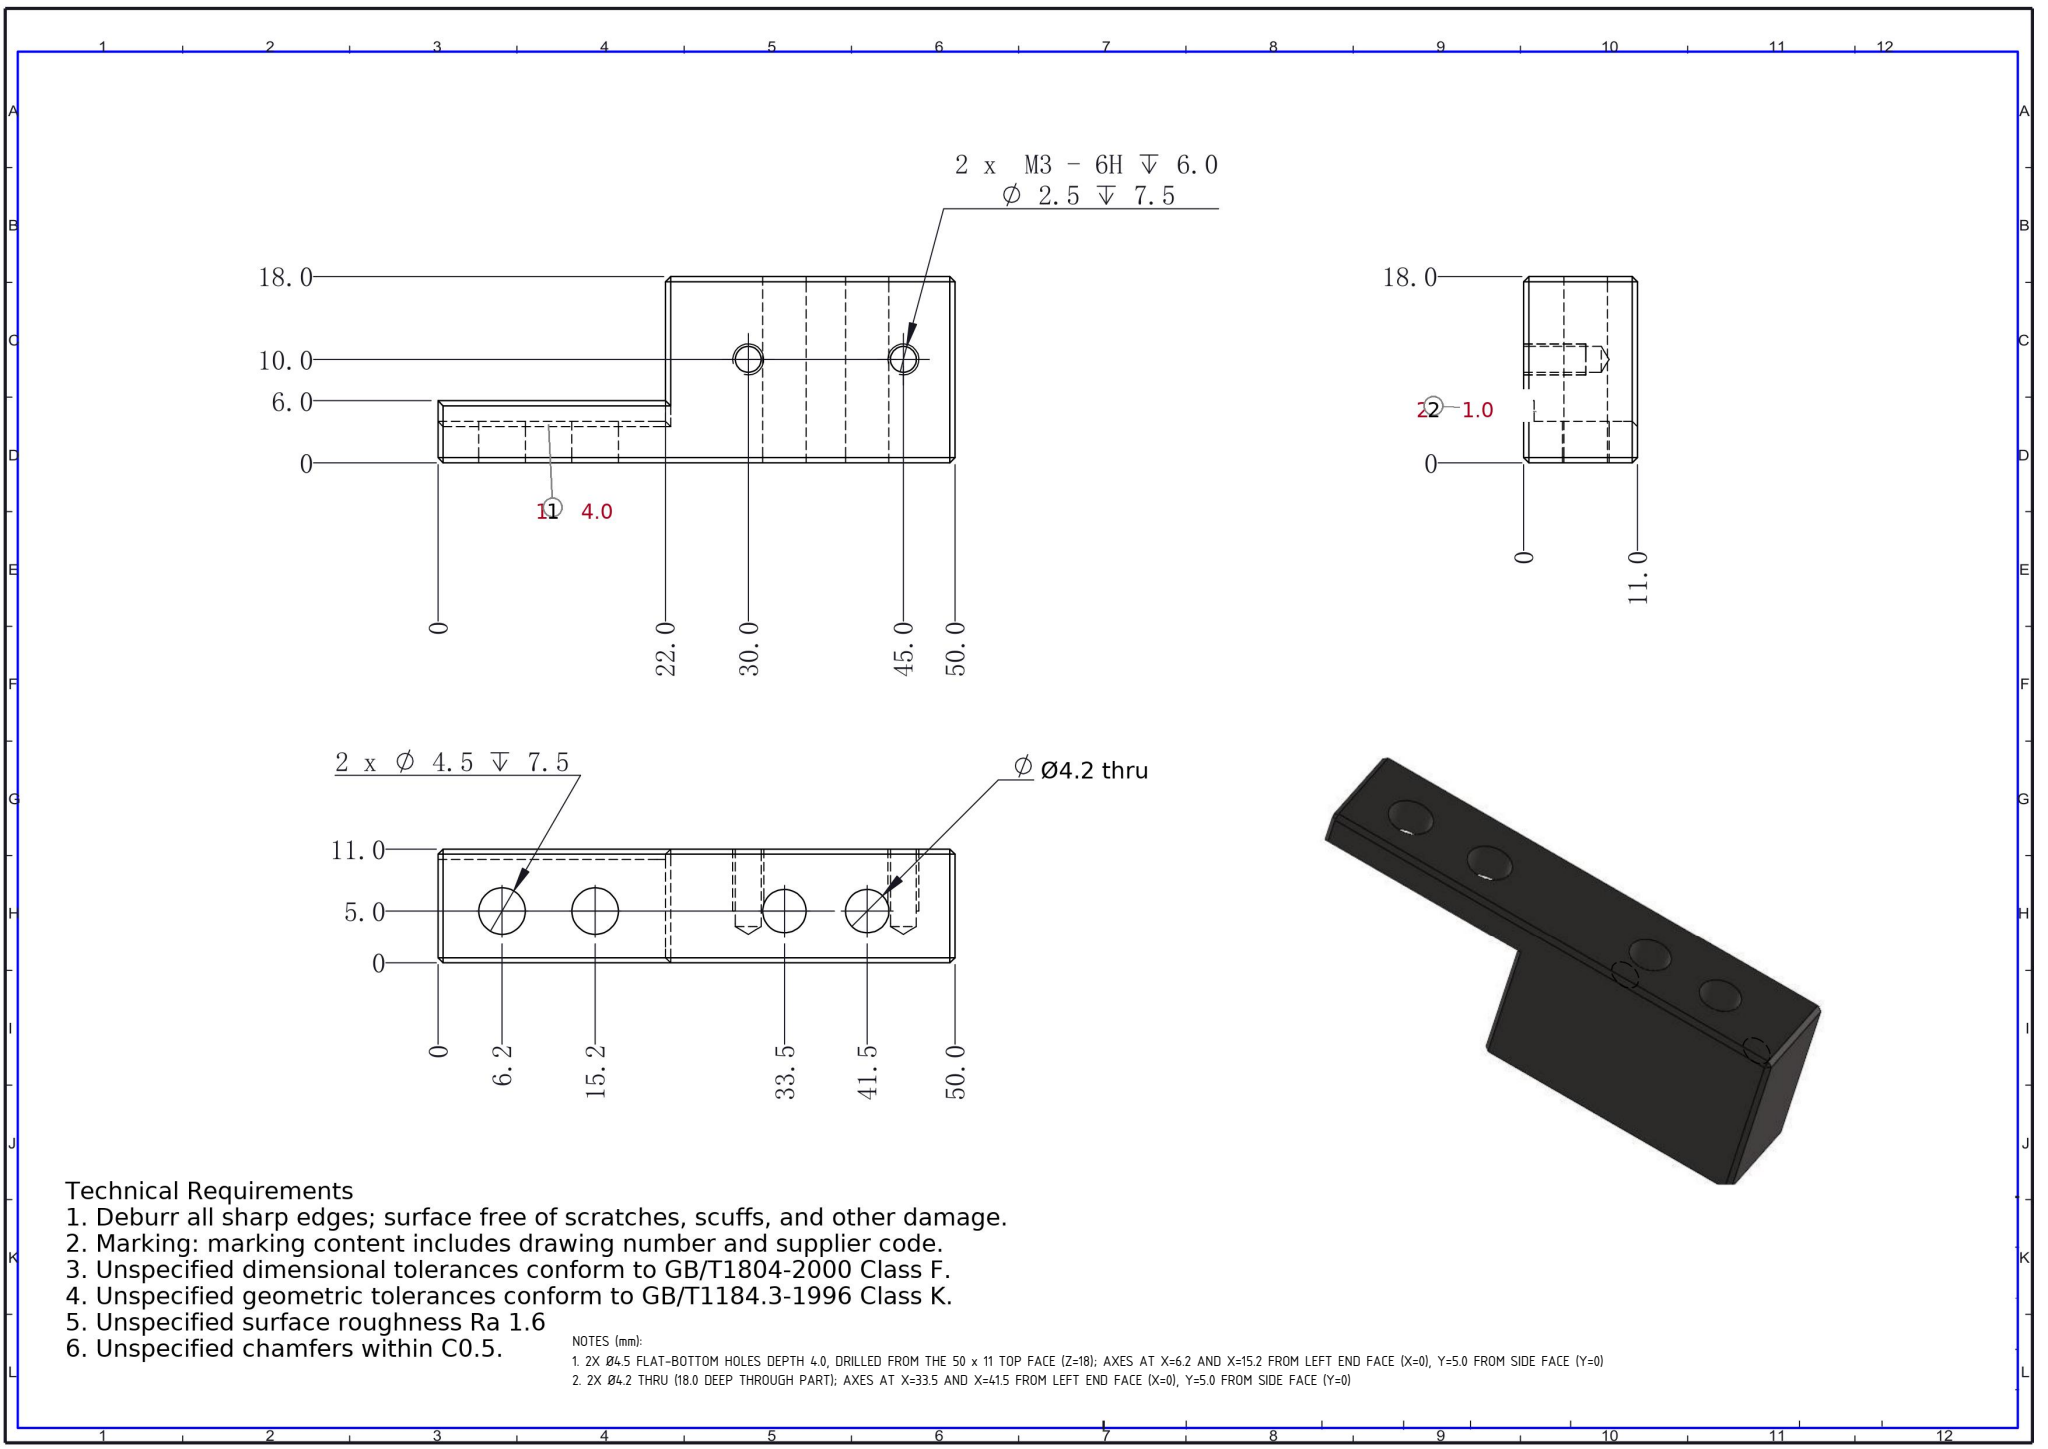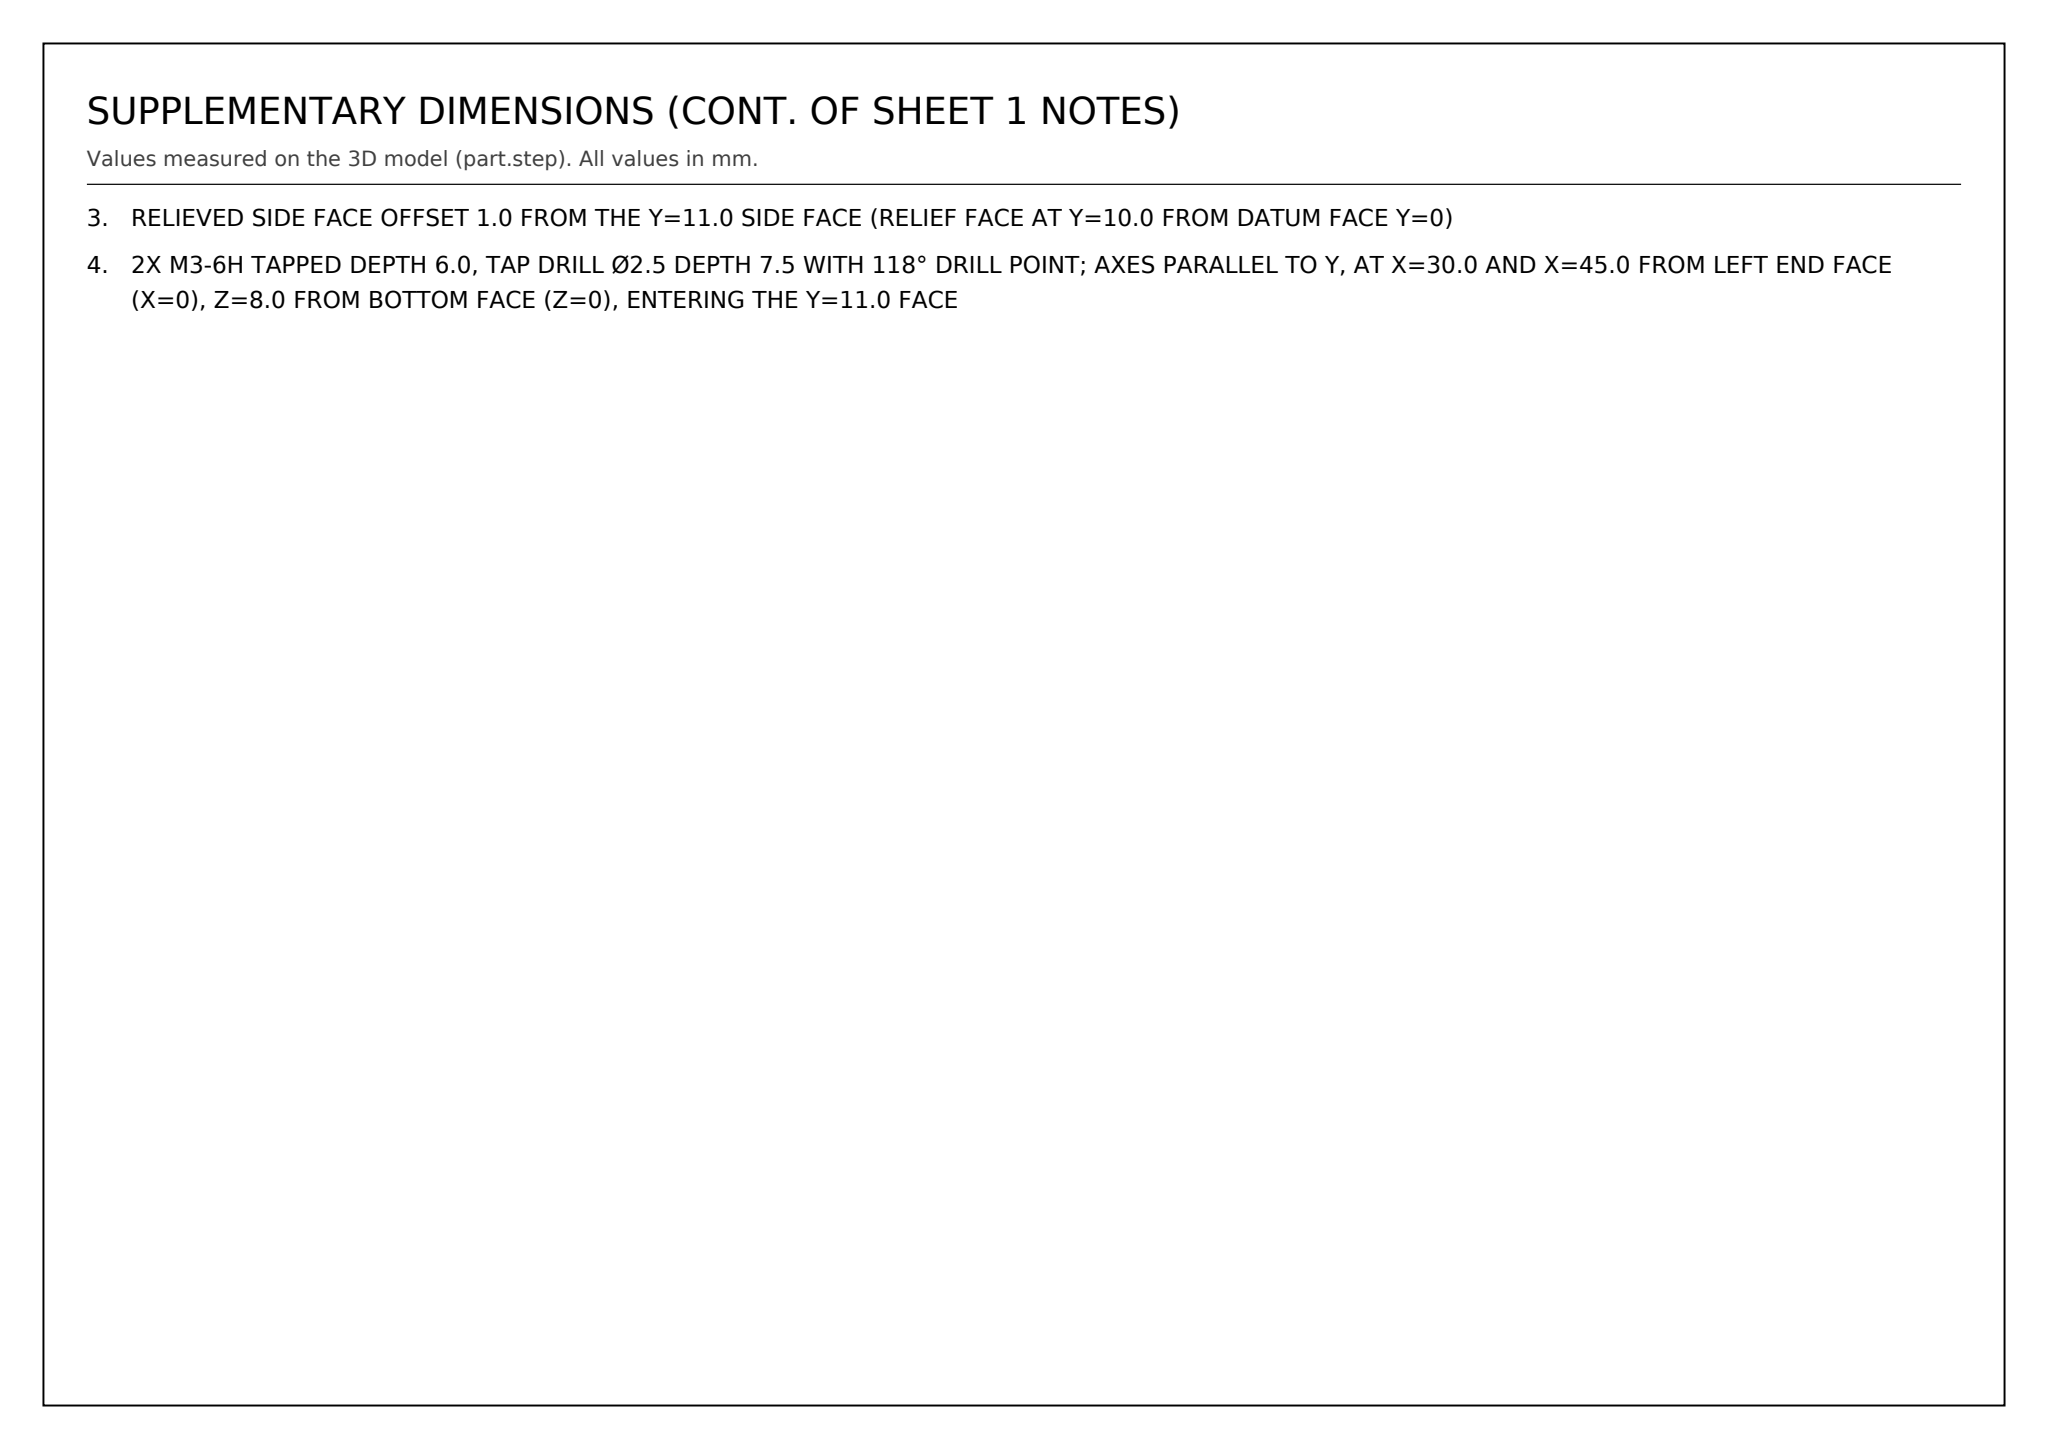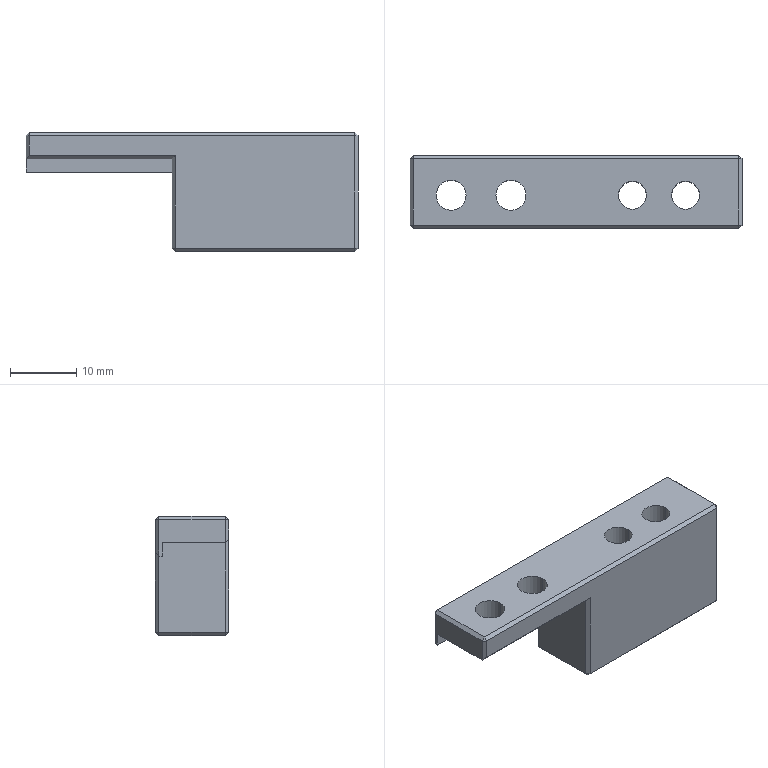Part | SolidWorks | mm | 1 solid | 50 faces | box 50 x 11 x 18 mm | volume 5815 mm3 | plane 34 | cylinder 12 | cone 4 | commonest cylinder face diameters 4.5 x4 2.5 x4 4.2 x4
Drawing notes:
2X Ø4.5 FLAT-BOTTOM HOLES DEPTH 4.0, DRILLED FROM THE 50 x 11 TOP FACE (Z=18); AXES AT X=6.2 AND X=15.2 FROM LEFT END FACE (X=0), Y=5.0 FROM SIDE FACE (Y=0) | from the solid: cylinders [4.5,"z",[6.2,5.0,null],4.0] and [4.5,"z",[15.2,5.0,null],4.0]; bbox_xyz z=18 with axis_plane z=14 (hole bottom)
2X Ø4.2 THRU (18.0 DEEP THROUGH PART); AXES AT X=33.5 AND X=41.5 FROM LEFT END FACE (X=0), Y=5.0 FROM SIDE FACE (Y=0) | from the solid: cylinders [4.2,"z",[33.5,5.0,null],18.0] and [4.2,"z",[41.5,5.0,null],18.0]; bbox z=18.0
RELIEVED SIDE FACE OFFSET 1.0 FROM THE Y=11.0 SIDE FACE (RELIEF FACE AT Y=10.0 FROM DATUM FACE Y=0) | from the solid: axis_planes y=10.0 and y=11.0; bbox_xyz y=11.0
2X M3-6H TAPPED DEPTH 6.0, TAP DRILL Ø2.5 DEPTH 7.5 WITH 118° DRILL POINT; AXES PARALLEL TO Y, AT X=30.0 AND X=45.0 FROM LEFT END FACE (X=0), Z=8.0 FROM BOTTOM FACE (Z=0), ENTERING THE Y=11.0 FACE | from the solid: cylinders [2.5,"y",[30.0,null,8.0],7.5] and [2.5,"y",[45.0,null,8.0],7.5]; cones [118.0,2.5]
build123d program:
from build123d import *

# Parameters (mm, degrees)
SKETCH1_W                = 50
SKETCH1_H                = 11
BOSS_EXTRUDE1_DEPTH      = 18
SKETCH2_W                = 22
SKETCH2_H                = 10
CUT_EXTRUDE1_DEPTH       = 14
SKETCH5_R                = 2.1
CUT_EXTRUDE3_DEPTH       = 19
M3_TAPPED_HOLE1_D        = 2.5
M3_TAPPED_HOLE1_DEPTH    = 7.5
M3_TAPPED_HOLE1_TIP      = 0.7511
SKETCH10_W               = 22
SKETCH10_H               = 12
CUT_EXTRUDE4_DEPTH       = 10
M4_CLEARANCE_HOLE1_D     = 4.5
M4_CLEARANCE_HOLE1_DEPTH = 7.5
M4_CLEARANCE_HOLE1_TIP   = 1.352
CHAMFER1_SIZE            = 0.5


with BuildPart() as part:
    # Sketch1 → Boss-Extrude1 (new body)
    with BuildSketch(Plane.XY):
        Rectangle(SKETCH1_W, SKETCH1_H)
    extrude(amount=BOSS_EXTRUDE1_DEPTH)

    # Sketch2 → Cut-Extrude1 (cut)
    with BuildSketch(Plane(origin=(0, 0, 0), x_dir=(-1, 0, 0), z_dir=(0, 0, -1))):
        with Locations((14, -0.5)):
            Rectangle(SKETCH2_W, SKETCH2_H)
    extrude(amount=-CUT_EXTRUDE1_DEPTH, mode=Mode.SUBTRACT)

    # Sketch5 → Cut-Extrude3 (cut)
    with BuildSketch(Plane.XY.offset(18)):
        with Locations((16.5, -0.5)):
            Circle(SKETCH5_R)
        with Locations((8.5, -0.5)):
            Circle(SKETCH5_R)
    extrude(amount=-CUT_EXTRUDE3_DEPTH, mode=Mode.SUBTRACT)

    # M3 Tapped Hole1
    with Locations(Plane(origin=(0, 5.5, 0), x_dir=(1, 0, 0), z_dir=(0, 1, 0))):
        with Locations((20, -8), (5, -8)):
            Hole(M3_TAPPED_HOLE1_D / 2, depth=M3_TAPPED_HOLE1_DEPTH)
            with Locations((0, 0, -(M3_TAPPED_HOLE1_DEPTH + M3_TAPPED_HOLE1_TIP / 2))):  # 118° drill point
                Cone(0, M3_TAPPED_HOLE1_D / 2, M3_TAPPED_HOLE1_TIP, mode=Mode.SUBTRACT)

    # Sketch10 → Cut-Extrude4 (cut)
    with BuildSketch(Plane(origin=(0, 5.5, 0), x_dir=(1, 0, 0), z_dir=(0, 1, 0))):
        with Locations((-14, -6)):
            Rectangle(SKETCH10_W, SKETCH10_H)
    extrude(amount=-CUT_EXTRUDE4_DEPTH, mode=Mode.SUBTRACT)

    # M4 Clearance Hole1
    with Locations(Plane.XY.offset(18)):
        with Locations((-9.8, -0.5), (-18.8, -0.5)):
            Hole(M4_CLEARANCE_HOLE1_D / 2, depth=M4_CLEARANCE_HOLE1_DEPTH)
            with Locations((0, 0, -(M4_CLEARANCE_HOLE1_DEPTH + M4_CLEARANCE_HOLE1_TIP / 2))):  # 118° drill point
                Cone(0, M4_CLEARANCE_HOLE1_D / 2, M4_CLEARANCE_HOLE1_TIP, mode=Mode.SUBTRACT)

    # Chamfer1
    chamfer1_edges = [part.edges().sort_by_distance(p)[0] for p in [
        (25, 0, 18),
        (11, -5.5, 0),
        (0, 5.5, 18),
        (-3, 0, 0),
        (-3, -5.5, 7),
        (-14, -5.5, 14),
        (-25, 0, 18),
        (11, 5.5, 0),
        (25, 0, 0),
        (-14, 5.5, 12),
        (-3, 5.5, 6),
        (-25, 5.5, 15),
        (25, 5.5, 9),
        (25, -5.5, 9),
        (-25, -5.5, 16),
        (0, -5.5, 18),
    ]]
    chamfer(chamfer1_edges, length=CHAMFER1_SIZE)


solid = part.part